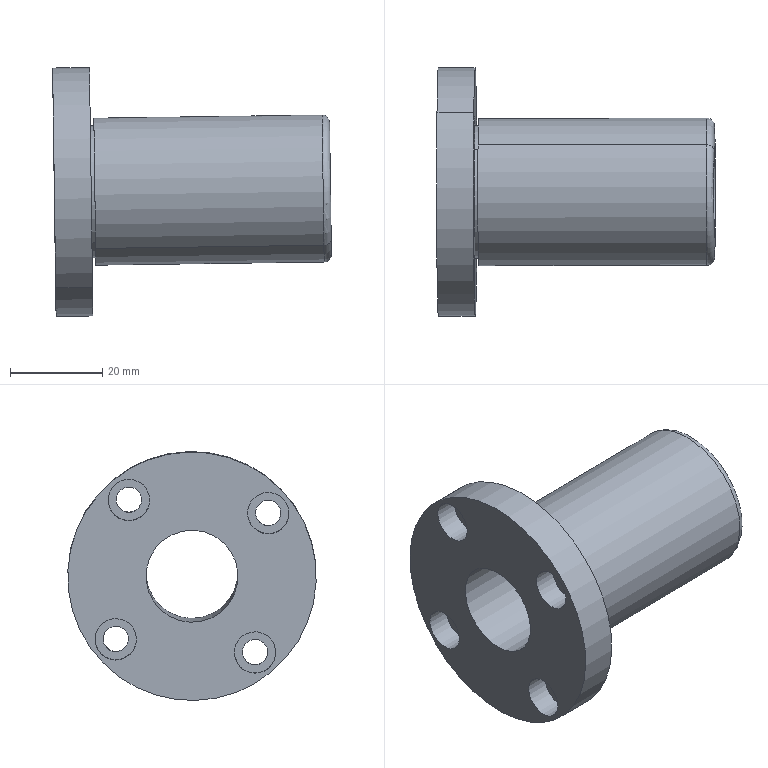Component | SolidWorks | DA-0220-LHFR20-1-15 | 1 solid | 34 faces | box 60.57 x 54 x 54.11 mm | volume 39543 mm3 | cylinder 24 | plane 8 | torus 2 | commonest cylinder face diameters 9 x8 5.5 x8 20 x2 28.8 x2 32 x2 54 x2
STEP:
#1=COLOUR_RGB('',0.7922,0.8196,0.9333);
#2=FILL_AREA_STYLE_COLOUR('',#1);
#3=FILL_AREA_STYLE('',(#2));
#4=SURFACE_STYLE_FILL_AREA(#3);
#5=SURFACE_SIDE_STYLE('',(#4));
#6=SURFACE_STYLE_USAGE(.BOTH.,#5);
#7=PRESENTATION_STYLE_ASSIGNMENT((#6));
#8=CARTESIAN_POINT('',(20.766,-3.293,-2.237));
#9=VERTEX_POINT('',#8);
#10=CARTESIAN_POINT('',(20.78,-4.096,-3.207));
#11=VERTEX_POINT('',#10);
#12=CARTESIAN_POINT('',(20.773,-3.694,-2.722));
#13=DIRECTION('',(-0.9999,-0.000404,-0.01395));
#14=DIRECTION('',(0.01101,-0.6374,-0.7704));
#15=AXIS2_PLACEMENT_3D('',#12,#13,#14);
#16=CIRCLE('',#15,0.6299);
#17=EDGE_CURVE('',#9,#11,#16,.T.);
#18=ORIENTED_EDGE('',*,*,#17,.F.);
#19=CARTESIAN_POINT('',(20.83,-3.333,-2.285));
#20=VERTEX_POINT('',#19);
#21=CARTESIAN_POINT('',(20.767,-3.333,-2.285));
#22=DIRECTION('',(0.008584,0.7705,-0.6374));
#23=DIRECTION('',(0.,0.6374,0.7705));
#24=AXIS2_PLACEMENT_3D('',#21,#22,#23);
#25=CIRCLE('',#24,0.06299);
#26=EDGE_CURVE('',#9,#20,#25,.T.);
#27=ORIENTED_EDGE('',*,*,#26,.T.);
#28=CARTESIAN_POINT('',(20.843,-4.056,-3.158));
#29=VERTEX_POINT('',#28);
#30=CARTESIAN_POINT('',(20.836,-3.694,-2.721));
#31=DIRECTION('',(0.9999,0.000404,0.01395));
#32=DIRECTION('',(0.01101,-0.6374,-0.7704));
#33=AXIS2_PLACEMENT_3D('',#30,#31,#32);
#34=CIRCLE('',#33,0.5669);
#35=EDGE_CURVE('',#29,#20,#34,.T.);
#36=ORIENTED_EDGE('',*,*,#35,.F.);
#37=CARTESIAN_POINT('',(20.78,-4.056,-3.159));
#38=DIRECTION('',(-0.008584,-0.7705,0.6374));
#39=DIRECTION('',(0.,-0.6374,-0.7705));
#40=AXIS2_PLACEMENT_3D('',#37,#38,#39);
#41=CIRCLE('',#40,0.06299);
#42=EDGE_CURVE('',#11,#29,#41,.T.);
#43=ORIENTED_EDGE('',*,*,#42,.F.);
#44=EDGE_LOOP('',(#18,#27,#36,#43));
#45=FACE_OUTER_BOUND('',#44,.T.);
#46=CARTESIAN_POINT('',(20.773,-3.694,-2.722));
#47=DIRECTION('',(0.9999,0.000404,0.01395));
#48=DIRECTION('',(0.01101,-0.6374,-0.7704));
#49=AXIS2_PLACEMENT_3D('',#46,#47,#48);
#50=TOROIDAL_SURFACE('',#49,0.5669,0.06299);
#51=ADVANCED_FACE('',(#45),#50,.T.);
#52=CARTESIAN_POINT('',(18.668,-3.269,-2.236));
#53=VERTEX_POINT('',#52);
#54=CARTESIAN_POINT('',(18.664,-3.043,-1.963));
#55=VERTEX_POINT('',#54);
#56=CARTESIAN_POINT('',(18.666,-3.156,-2.099));
#57=DIRECTION('',(-0.9999,-0.000404,-0.01395));
#58=DIRECTION('',(-0.01101,0.6374,0.7704));
#59=AXIS2_PLACEMENT_3D('',#56,#57,#58);
#60=CIRCLE('',#59,0.1772);
#61=EDGE_CURVE('',#53,#55,#60,.T.);
#62=ORIENTED_EDGE('',*,*,#61,.F.);
#63=CARTESIAN_POINT('',(18.467,-3.269,-2.239));
#64=VERTEX_POINT('',#63);
#65=CARTESIAN_POINT('',(18.467,-3.269,-2.239));
#66=DIRECTION('',(-0.9999,-0.000404,-0.01395));
#67=VECTOR('',#66,39.37);
#68=LINE('',#65,#67);
#69=EDGE_CURVE('',#53,#64,#68,.T.);
#70=ORIENTED_EDGE('',*,*,#69,.T.);
#71=CARTESIAN_POINT('',(18.463,-3.043,-1.966));
#72=VERTEX_POINT('',#71);
#73=CARTESIAN_POINT('',(18.465,-3.156,-2.102));
#74=DIRECTION('',(-0.9999,-0.000404,-0.01395));
#75=DIRECTION('',(-0.01101,0.6374,0.7704));
#76=AXIS2_PLACEMENT_3D('',#73,#74,#75);
#77=CIRCLE('',#76,0.1772);
#78=EDGE_CURVE('',#64,#72,#77,.T.);
#79=ORIENTED_EDGE('',*,*,#78,.T.);
#80=CARTESIAN_POINT('',(18.463,-3.043,-1.966));
#81=DIRECTION('',(-0.9999,-0.000404,-0.01395));
#82=VECTOR('',#81,39.37);
#83=LINE('',#80,#82);
#84=EDGE_CURVE('',#55,#72,#83,.T.);
#85=ORIENTED_EDGE('',*,*,#84,.F.);
#86=EDGE_LOOP('',(#62,#70,#79,#85));
#87=FACE_OUTER_BOUND('',#86,.T.);
#88=CARTESIAN_POINT('',(18.465,-3.156,-2.102));
#89=DIRECTION('',(-0.9999,-0.000404,-0.01395));
#90=DIRECTION('',(-0.01101,0.6374,0.7704));
#91=AXIS2_PLACEMENT_3D('',#88,#89,#90);
#92=CYLINDRICAL_SURFACE('',#91,0.1772);
#93=ADVANCED_FACE('',(#87),#92,.F.);
#94=CARTESIAN_POINT('',(18.779,-3.087,-2.014));
#95=VERTEX_POINT('',#94);
#96=CARTESIAN_POINT('',(18.781,-3.225,-2.181));
#97=VERTEX_POINT('',#96);
#98=CARTESIAN_POINT('',(18.78,-3.156,-2.098));
#99=DIRECTION('',(0.9999,0.000404,0.01395));
#100=DIRECTION('',(0.01101,-0.6374,-0.7704));
#101=AXIS2_PLACEMENT_3D('',#98,#99,#100);
#102=CIRCLE('',#101,0.1083);
#103=EDGE_CURVE('',#95,#97,#102,.T.);
#104=ORIENTED_EDGE('',*,*,#103,.T.);
#105=CARTESIAN_POINT('',(18.667,-3.225,-2.183));
#106=VERTEX_POINT('',#105);
#107=CARTESIAN_POINT('',(18.466,-3.225,-2.186));
#108=DIRECTION('',(-0.9999,-0.000404,-0.01395));
#109=VECTOR('',#108,39.37);
#110=LINE('',#107,#109);
#111=EDGE_CURVE('',#97,#106,#110,.T.);
#112=ORIENTED_EDGE('',*,*,#111,.T.);
#113=CARTESIAN_POINT('',(18.665,-3.087,-2.016));
#114=VERTEX_POINT('',#113);
#115=CARTESIAN_POINT('',(18.666,-3.156,-2.099));
#116=DIRECTION('',(-0.9999,-0.000404,-0.01395));
#117=DIRECTION('',(-0.01101,0.6374,0.7704));
#118=AXIS2_PLACEMENT_3D('',#115,#116,#117);
#119=CIRCLE('',#118,0.1083);
#120=EDGE_CURVE('',#106,#114,#119,.T.);
#121=ORIENTED_EDGE('',*,*,#120,.T.);
#122=CARTESIAN_POINT('',(18.464,-3.087,-2.019));
#123=DIRECTION('',(-0.9999,-0.000404,-0.01395));
#124=VECTOR('',#123,39.37);
#125=LINE('',#122,#124);
#126=EDGE_CURVE('',#95,#114,#125,.T.);
#127=ORIENTED_EDGE('',*,*,#126,.F.);
#128=EDGE_LOOP('',(#104,#112,#121,#127));
#129=FACE_OUTER_BOUND('',#128,.T.);
#130=CARTESIAN_POINT('',(18.465,-3.156,-2.102));
#131=DIRECTION('',(-0.9999,-0.000404,-0.01395));
#132=DIRECTION('',(-0.01101,0.6374,0.7704));
#133=AXIS2_PLACEMENT_3D('',#130,#131,#132);
#134=CYLINDRICAL_SURFACE('',#133,0.1083);
#135=ADVANCED_FACE('',(#129),#134,.F.);
#136=CARTESIAN_POINT('',(18.67,-4.46,-2.348));
#137=VERTEX_POINT('',#136);
#138=CARTESIAN_POINT('',(18.666,-4.235,-2.075));
#139=VERTEX_POINT('',#138);
#140=CARTESIAN_POINT('',(18.668,-4.348,-2.212));
#141=DIRECTION('',(-0.9999,-0.000404,-0.01395));
#142=DIRECTION('',(-0.01101,0.6374,0.7704));
#143=AXIS2_PLACEMENT_3D('',#140,#141,#142);
#144=CIRCLE('',#143,0.1772);
#145=EDGE_CURVE('',#137,#139,#144,.T.);
#146=ORIENTED_EDGE('',*,*,#145,.F.);
#147=CARTESIAN_POINT('',(18.469,-4.461,-2.351));
#148=VERTEX_POINT('',#147);
#149=CARTESIAN_POINT('',(18.469,-4.461,-2.351));
#150=DIRECTION('',(-0.9999,-0.000404,-0.01395));
#151=VECTOR('',#150,39.37);
#152=LINE('',#149,#151);
#153=EDGE_CURVE('',#137,#148,#152,.T.);
#154=ORIENTED_EDGE('',*,*,#153,.T.);
#155=CARTESIAN_POINT('',(18.465,-4.235,-2.078));
#156=VERTEX_POINT('',#155);
#157=CARTESIAN_POINT('',(18.467,-4.348,-2.215));
#158=DIRECTION('',(-0.9999,-0.000404,-0.01395));
#159=DIRECTION('',(-0.01101,0.6374,0.7704));
#160=AXIS2_PLACEMENT_3D('',#157,#158,#159);
#161=CIRCLE('',#160,0.1772);
#162=EDGE_CURVE('',#148,#156,#161,.T.);
#163=ORIENTED_EDGE('',*,*,#162,.T.);
#164=CARTESIAN_POINT('',(18.465,-4.235,-2.078));
#165=DIRECTION('',(-0.9999,-0.000404,-0.01395));
#166=VECTOR('',#165,39.37);
#167=LINE('',#164,#166);
#168=EDGE_CURVE('',#139,#156,#167,.T.);
#169=ORIENTED_EDGE('',*,*,#168,.F.);
#170=EDGE_LOOP('',(#146,#154,#163,#169));
#171=FACE_OUTER_BOUND('',#170,.T.);
#172=CARTESIAN_POINT('',(18.467,-4.348,-2.215));
#173=DIRECTION('',(-0.9999,-0.000404,-0.01395));
#174=DIRECTION('',(-0.01101,0.6374,0.7704));
#175=AXIS2_PLACEMENT_3D('',#172,#173,#174);
#176=CYLINDRICAL_SURFACE('',#175,0.1772);
#177=ADVANCED_FACE('',(#171),#176,.F.);
#178=CARTESIAN_POINT('',(18.781,-4.278,-2.127));
#179=VERTEX_POINT('',#178);
#180=CARTESIAN_POINT('',(18.783,-4.416,-2.294));
#181=VERTEX_POINT('',#180);
#182=CARTESIAN_POINT('',(18.782,-4.347,-2.21));
#183=DIRECTION('',(0.9999,0.000404,0.01395));
#184=DIRECTION('',(0.01101,-0.6374,-0.7704));
#185=AXIS2_PLACEMENT_3D('',#182,#183,#184);
#186=CIRCLE('',#185,0.1083);
#187=EDGE_CURVE('',#179,#181,#186,.T.);
#188=ORIENTED_EDGE('',*,*,#187,.T.);
#189=CARTESIAN_POINT('',(18.669,-4.417,-2.295));
#190=VERTEX_POINT('',#189);
#191=CARTESIAN_POINT('',(18.468,-4.417,-2.298));
#192=DIRECTION('',(-0.9999,-0.000404,-0.01395));
#193=VECTOR('',#192,39.37);
#194=LINE('',#191,#193);
#195=EDGE_CURVE('',#181,#190,#194,.T.);
#196=ORIENTED_EDGE('',*,*,#195,.T.);
#197=CARTESIAN_POINT('',(18.667,-4.278,-2.129));
#198=VERTEX_POINT('',#197);
#199=CARTESIAN_POINT('',(18.668,-4.348,-2.212));
#200=DIRECTION('',(-0.9999,-0.000404,-0.01395));
#201=DIRECTION('',(-0.01101,0.6374,0.7704));
#202=AXIS2_PLACEMENT_3D('',#199,#200,#201);
#203=CIRCLE('',#202,0.1083);
#204=EDGE_CURVE('',#190,#198,#203,.T.);
#205=ORIENTED_EDGE('',*,*,#204,.T.);
#206=CARTESIAN_POINT('',(18.466,-4.279,-2.131));
#207=DIRECTION('',(-0.9999,-0.000404,-0.01395));
#208=VECTOR('',#207,39.37);
#209=LINE('',#206,#208);
#210=EDGE_CURVE('',#179,#198,#209,.T.);
#211=ORIENTED_EDGE('',*,*,#210,.F.);
#212=EDGE_LOOP('',(#188,#196,#205,#211));
#213=FACE_OUTER_BOUND('',#212,.T.);
#214=CARTESIAN_POINT('',(18.467,-4.348,-2.215));
#215=DIRECTION('',(-0.9999,-0.000404,-0.01395));
#216=DIRECTION('',(-0.01101,0.6374,0.7704));
#217=AXIS2_PLACEMENT_3D('',#214,#215,#216);
#218=CYLINDRICAL_SURFACE('',#217,0.1083);
#219=ADVANCED_FACE('',(#213),#218,.F.);
#220=CARTESIAN_POINT('',(18.686,-4.348,-3.54));
#221=VERTEX_POINT('',#220);
#222=CARTESIAN_POINT('',(18.683,-4.122,-3.267));
#223=VERTEX_POINT('',#222);
#224=CARTESIAN_POINT('',(18.685,-4.235,-3.404));
#225=DIRECTION('',(-0.9999,-0.000404,-0.01395));
#226=DIRECTION('',(-0.01101,0.6374,0.7704));
#227=AXIS2_PLACEMENT_3D('',#224,#225,#226);
#228=CIRCLE('',#227,0.1772);
#229=EDGE_CURVE('',#221,#223,#228,.T.);
#230=ORIENTED_EDGE('',*,*,#229,.F.);
#231=CARTESIAN_POINT('',(18.486,-4.348,-3.543));
#232=VERTEX_POINT('',#231);
#233=CARTESIAN_POINT('',(18.486,-4.348,-3.543));
#234=DIRECTION('',(-0.9999,-0.000404,-0.01395));
#235=VECTOR('',#234,39.37);
#236=LINE('',#233,#235);
#237=EDGE_CURVE('',#221,#232,#236,.T.);
#238=ORIENTED_EDGE('',*,*,#237,.T.);
#239=CARTESIAN_POINT('',(18.482,-4.122,-3.27));
#240=VERTEX_POINT('',#239);
#241=CARTESIAN_POINT('',(18.484,-4.235,-3.406));
#242=DIRECTION('',(-0.9999,-0.000404,-0.01395));
#243=DIRECTION('',(-0.01101,0.6374,0.7704));
#244=AXIS2_PLACEMENT_3D('',#241,#242,#243);
#245=CIRCLE('',#244,0.1772);
#246=EDGE_CURVE('',#232,#240,#245,.T.);
#247=ORIENTED_EDGE('',*,*,#246,.T.);
#248=CARTESIAN_POINT('',(18.482,-4.122,-3.27));
#249=DIRECTION('',(-0.9999,-0.000404,-0.01395));
#250=VECTOR('',#249,39.37);
#251=LINE('',#248,#250);
#252=EDGE_CURVE('',#223,#240,#251,.T.);
#253=ORIENTED_EDGE('',*,*,#252,.F.);
#254=EDGE_LOOP('',(#230,#238,#247,#253));
#255=FACE_OUTER_BOUND('',#254,.T.);
#256=CARTESIAN_POINT('',(18.484,-4.235,-3.406));
#257=DIRECTION('',(-0.9999,-0.000404,-0.01395));
#258=DIRECTION('',(-0.01101,0.6374,0.7704));
#259=AXIS2_PLACEMENT_3D('',#256,#257,#258);
#260=CYLINDRICAL_SURFACE('',#259,0.1772);
#261=ADVANCED_FACE('',(#255),#260,.F.);
#262=CARTESIAN_POINT('',(18.797,-4.166,-3.319));
#263=VERTEX_POINT('',#262);
#264=CARTESIAN_POINT('',(18.8,-4.304,-3.485));
#265=VERTEX_POINT('',#264);
#266=CARTESIAN_POINT('',(18.799,-4.235,-3.402));
#267=DIRECTION('',(0.9999,0.000404,0.01395));
#268=DIRECTION('',(0.01101,-0.6374,-0.7704));
#269=AXIS2_PLACEMENT_3D('',#266,#267,#268);
#270=CIRCLE('',#269,0.1083);
#271=EDGE_CURVE('',#263,#265,#270,.T.);
#272=ORIENTED_EDGE('',*,*,#271,.T.);
#273=CARTESIAN_POINT('',(18.686,-4.304,-3.487));
#274=VERTEX_POINT('',#273);
#275=CARTESIAN_POINT('',(18.485,-4.304,-3.49));
#276=DIRECTION('',(-0.9999,-0.000404,-0.01395));
#277=VECTOR('',#276,39.37);
#278=LINE('',#275,#277);
#279=EDGE_CURVE('',#265,#274,#278,.T.);
#280=ORIENTED_EDGE('',*,*,#279,.T.);
#281=CARTESIAN_POINT('',(18.683,-4.166,-3.32));
#282=VERTEX_POINT('',#281);
#283=CARTESIAN_POINT('',(18.685,-4.235,-3.404));
#284=DIRECTION('',(-0.9999,-0.000404,-0.01395));
#285=DIRECTION('',(-0.01101,0.6374,0.7704));
#286=AXIS2_PLACEMENT_3D('',#283,#284,#285);
#287=CIRCLE('',#286,0.1083);
#288=EDGE_CURVE('',#274,#282,#287,.T.);
#289=ORIENTED_EDGE('',*,*,#288,.T.);
#290=CARTESIAN_POINT('',(18.483,-4.166,-3.323));
#291=DIRECTION('',(-0.9999,-0.000404,-0.01395));
#292=VECTOR('',#291,39.37);
#293=LINE('',#290,#292);
#294=EDGE_CURVE('',#263,#282,#293,.T.);
#295=ORIENTED_EDGE('',*,*,#294,.F.);
#296=EDGE_LOOP('',(#272,#280,#289,#295));
#297=FACE_OUTER_BOUND('',#296,.T.);
#298=CARTESIAN_POINT('',(18.484,-4.235,-3.406));
#299=DIRECTION('',(-0.9999,-0.000404,-0.01395));
#300=DIRECTION('',(-0.01101,0.6374,0.7704));
#301=AXIS2_PLACEMENT_3D('',#298,#299,#300);
#302=CYLINDRICAL_SURFACE('',#301,0.1083);
#303=ADVANCED_FACE('',(#297),#302,.F.);
#304=CARTESIAN_POINT('',(18.684,-3.156,-3.427));
#305=VERTEX_POINT('',#304);
#306=CARTESIAN_POINT('',(18.681,-2.93,-3.154));
#307=VERTEX_POINT('',#306);
#308=CARTESIAN_POINT('',(18.682,-3.043,-3.291));
#309=DIRECTION('',(-0.9999,-0.000404,-0.01395));
#310=DIRECTION('',(-0.01101,0.6374,0.7704));
#311=AXIS2_PLACEMENT_3D('',#308,#309,#310);
#312=CIRCLE('',#311,0.1772);
#313=EDGE_CURVE('',#305,#307,#312,.T.);
#314=ORIENTED_EDGE('',*,*,#313,.F.);
#315=CARTESIAN_POINT('',(18.484,-3.156,-3.43));
#316=VERTEX_POINT('',#315);
#317=CARTESIAN_POINT('',(18.484,-3.156,-3.43));
#318=DIRECTION('',(-0.9999,-0.000404,-0.01395));
#319=VECTOR('',#318,39.37);
#320=LINE('',#317,#319);
#321=EDGE_CURVE('',#305,#316,#320,.T.);
#322=ORIENTED_EDGE('',*,*,#321,.T.);
#323=CARTESIAN_POINT('',(18.48,-2.93,-3.157));
#324=VERTEX_POINT('',#323);
#325=CARTESIAN_POINT('',(18.482,-3.043,-3.294));
#326=DIRECTION('',(-0.9999,-0.000404,-0.01395));
#327=DIRECTION('',(-0.01101,0.6374,0.7704));
#328=AXIS2_PLACEMENT_3D('',#325,#326,#327);
#329=CIRCLE('',#328,0.1772);
#330=EDGE_CURVE('',#316,#324,#329,.T.);
#331=ORIENTED_EDGE('',*,*,#330,.T.);
#332=CARTESIAN_POINT('',(18.48,-2.93,-3.157));
#333=DIRECTION('',(-0.9999,-0.000404,-0.01395));
#334=VECTOR('',#333,39.37);
#335=LINE('',#332,#334);
#336=EDGE_CURVE('',#307,#324,#335,.T.);
#337=ORIENTED_EDGE('',*,*,#336,.F.);
#338=EDGE_LOOP('',(#314,#322,#331,#337));
#339=FACE_OUTER_BOUND('',#338,.T.);
#340=CARTESIAN_POINT('',(18.482,-3.043,-3.294));
#341=DIRECTION('',(-0.9999,-0.000404,-0.01395));
#342=DIRECTION('',(-0.01101,0.6374,0.7704));
#343=AXIS2_PLACEMENT_3D('',#340,#341,#342);
#344=CYLINDRICAL_SURFACE('',#343,0.1772);
#345=ADVANCED_FACE('',(#339),#344,.F.);
#346=CARTESIAN_POINT('',(18.795,-2.974,-3.206));
#347=VERTEX_POINT('',#346);
#348=CARTESIAN_POINT('',(18.798,-3.112,-3.373));
#349=VERTEX_POINT('',#348);
#350=CARTESIAN_POINT('',(18.797,-3.043,-3.289));
#351=DIRECTION('',(0.9999,0.000404,0.01395));
#352=DIRECTION('',(0.01101,-0.6374,-0.7704));
#353=AXIS2_PLACEMENT_3D('',#350,#351,#352);
#354=CIRCLE('',#353,0.1083);
#355=EDGE_CURVE('',#347,#349,#354,.T.);
#356=ORIENTED_EDGE('',*,*,#355,.T.);
#357=CARTESIAN_POINT('',(18.684,-3.112,-3.374));
#358=VERTEX_POINT('',#357);
#359=CARTESIAN_POINT('',(18.483,-3.112,-3.377));
#360=DIRECTION('',(-0.9999,-0.000404,-0.01395));
#361=VECTOR('',#360,39.37);
#362=LINE('',#359,#361);
#363=EDGE_CURVE('',#349,#358,#362,.T.);
#364=ORIENTED_EDGE('',*,*,#363,.T.);
#365=CARTESIAN_POINT('',(18.681,-2.974,-3.208));
#366=VERTEX_POINT('',#365);
#367=CARTESIAN_POINT('',(18.682,-3.043,-3.291));
#368=DIRECTION('',(-0.9999,-0.000404,-0.01395));
#369=DIRECTION('',(-0.01101,0.6374,0.7704));
#370=AXIS2_PLACEMENT_3D('',#367,#368,#369);
#371=CIRCLE('',#370,0.1083);
#372=EDGE_CURVE('',#358,#366,#371,.T.);
#373=ORIENTED_EDGE('',*,*,#372,.T.);
#374=CARTESIAN_POINT('',(18.481,-2.974,-3.21));
#375=DIRECTION('',(-0.9999,-0.000404,-0.01395));
#376=VECTOR('',#375,39.37);
#377=LINE('',#374,#376);
#378=EDGE_CURVE('',#347,#366,#377,.T.);
#379=ORIENTED_EDGE('',*,*,#378,.F.);
#380=EDGE_LOOP('',(#356,#364,#373,#379));
#381=FACE_OUTER_BOUND('',#380,.T.);
#382=CARTESIAN_POINT('',(18.482,-3.043,-3.294));
#383=DIRECTION('',(-0.9999,-0.000404,-0.01395));
#384=DIRECTION('',(-0.01101,0.6374,0.7704));
#385=AXIS2_PLACEMENT_3D('',#382,#383,#384);
#386=CYLINDRICAL_SURFACE('',#385,0.1083);
#387=ADVANCED_FACE('',(#381),#386,.F.);
#388=CARTESIAN_POINT('',(20.841,-3.945,-3.025));
#389=VERTEX_POINT('',#388);
#390=CARTESIAN_POINT('',(20.832,-3.443,-2.418));
#391=VERTEX_POINT('',#390);
#392=CARTESIAN_POINT('',(20.836,-3.694,-2.721));
#393=DIRECTION('',(-0.9999,-0.000404,-0.01395));
#394=DIRECTION('',(-0.01101,0.6374,0.7704));
#395=AXIS2_PLACEMENT_3D('',#392,#393,#394);
#396=CIRCLE('',#395,0.3937);
#397=EDGE_CURVE('',#389,#391,#396,.T.);
#398=ORIENTED_EDGE('',*,*,#397,.F.);
#399=CARTESIAN_POINT('',(18.479,-3.946,-3.058));
#400=VERTEX_POINT('',#399);
#401=CARTESIAN_POINT('',(18.479,-3.946,-3.058));
#402=DIRECTION('',(-0.9999,-0.000404,-0.01395));
#403=VECTOR('',#402,39.37);
#404=LINE('',#401,#403);
#405=EDGE_CURVE('',#389,#400,#404,.T.);
#406=ORIENTED_EDGE('',*,*,#405,.T.);
#407=CARTESIAN_POINT('',(18.47,-3.444,-2.451));
#408=VERTEX_POINT('',#407);
#409=CARTESIAN_POINT('',(18.474,-3.695,-2.754));
#410=DIRECTION('',(-0.9999,-0.000404,-0.01395));
#411=DIRECTION('',(-0.01101,0.6374,0.7704));
#412=AXIS2_PLACEMENT_3D('',#409,#410,#411);
#413=CIRCLE('',#412,0.3937);
#414=EDGE_CURVE('',#400,#408,#413,.T.);
#415=ORIENTED_EDGE('',*,*,#414,.T.);
#416=CARTESIAN_POINT('',(18.47,-3.444,-2.451));
#417=DIRECTION('',(-0.9999,-0.000404,-0.01395));
#418=VECTOR('',#417,39.37);
#419=LINE('',#416,#418);
#420=EDGE_CURVE('',#391,#408,#419,.T.);
#421=ORIENTED_EDGE('',*,*,#420,.F.);
#422=EDGE_LOOP('',(#398,#406,#415,#421));
#423=FACE_OUTER_BOUND('',#422,.T.);
#424=CARTESIAN_POINT('',(18.474,-3.695,-2.754));
#425=DIRECTION('',(-0.9999,-0.000404,-0.01395));
#426=DIRECTION('',(-0.01101,0.6374,0.7704));
#427=AXIS2_PLACEMENT_3D('',#424,#425,#426);
#428=CYLINDRICAL_SURFACE('',#427,0.3937);
#429=ADVANCED_FACE('',(#423),#428,.F.);
#430=CARTESIAN_POINT('',(18.796,-4.057,-3.187));
#431=VERTEX_POINT('',#430);
#432=CARTESIAN_POINT('',(18.783,-3.334,-2.313));
#433=VERTEX_POINT('',#432);
#434=CARTESIAN_POINT('',(18.789,-3.695,-2.75));
#435=DIRECTION('',(0.9999,0.000404,0.01395));
#436=DIRECTION('',(0.01101,-0.6374,-0.7704));
#437=AXIS2_PLACEMENT_3D('',#434,#435,#436);
#438=CIRCLE('',#437,0.5669);
#439=EDGE_CURVE('',#431,#433,#438,.T.);
#440=ORIENTED_EDGE('',*,*,#439,.T.);
#441=CARTESIAN_POINT('',(18.815,-3.334,-2.313));
#442=VERTEX_POINT('',#441);
#443=CARTESIAN_POINT('',(18.468,-3.334,-2.317));
#444=DIRECTION('',(0.9999,0.000404,0.01395));
#445=VECTOR('',#444,39.37);
#446=LINE('',#443,#445);
#447=EDGE_CURVE('',#433,#442,#446,.T.);
#448=ORIENTED_EDGE('',*,*,#447,.T.);
#449=CARTESIAN_POINT('',(18.827,-4.057,-3.186));
#450=VERTEX_POINT('',#449);
#451=CARTESIAN_POINT('',(18.821,-3.695,-2.749));
#452=DIRECTION('',(0.9999,0.000404,0.01395));
#453=DIRECTION('',(0.01101,-0.6374,-0.7704));
#454=AXIS2_PLACEMENT_3D('',#451,#452,#453);
#455=CIRCLE('',#454,0.5669);
#456=EDGE_CURVE('',#450,#442,#455,.T.);
#457=ORIENTED_EDGE('',*,*,#456,.F.);
#458=CARTESIAN_POINT('',(18.481,-4.057,-3.191));
#459=DIRECTION('',(0.9999,0.000404,0.01395));
#460=VECTOR('',#459,39.37);
#461=LINE('',#458,#460);
#462=EDGE_CURVE('',#431,#450,#461,.T.);
#463=ORIENTED_EDGE('',*,*,#462,.F.);
#464=EDGE_LOOP('',(#440,#448,#457,#463));
#465=FACE_OUTER_BOUND('',#464,.T.);
#466=CARTESIAN_POINT('',(18.474,-3.695,-2.754));
#467=DIRECTION('',(0.9999,0.000404,0.01395));
#468=DIRECTION('',(0.01101,-0.6374,-0.7704));
#469=AXIS2_PLACEMENT_3D('',#466,#467,#468);
#470=CYLINDRICAL_SURFACE('',#469,0.5669);
#471=ADVANCED_FACE('',(#465),#470,.T.);
#472=CARTESIAN_POINT('',(18.828,-4.097,-3.235));
#473=VERTEX_POINT('',#472);
#474=CARTESIAN_POINT('',(18.814,-3.294,-2.264));
#475=VERTEX_POINT('',#474);
#476=CARTESIAN_POINT('',(18.821,-3.695,-2.749));
#477=DIRECTION('',(0.9999,0.000404,0.01395));
#478=DIRECTION('',(0.01101,-0.6374,-0.7704));
#479=AXIS2_PLACEMENT_3D('',#476,#477,#478);
#480=CIRCLE('',#479,0.6299);
#481=EDGE_CURVE('',#473,#475,#480,.T.);
#482=ORIENTED_EDGE('',*,*,#481,.T.);
#483=CARTESIAN_POINT('',(18.468,-3.294,-2.269));
#484=DIRECTION('',(0.9999,0.000404,0.01395));
#485=VECTOR('',#484,39.37);
#486=LINE('',#483,#485);
#487=EDGE_CURVE('',#475,#9,#486,.T.);
#488=ORIENTED_EDGE('',*,*,#487,.T.);
#489=ORIENTED_EDGE('',*,*,#17,.T.);
#490=CARTESIAN_POINT('',(18.481,-4.097,-3.24));
#491=DIRECTION('',(0.9999,0.000404,0.01395));
#492=VECTOR('',#491,39.37);
#493=LINE('',#490,#492);
#494=EDGE_CURVE('',#473,#11,#493,.T.);
#495=ORIENTED_EDGE('',*,*,#494,.F.);
#496=EDGE_LOOP('',(#482,#488,#489,#495));
#497=FACE_OUTER_BOUND('',#496,.T.);
#498=CARTESIAN_POINT('',(18.474,-3.695,-2.754));
#499=DIRECTION('',(0.9999,0.000404,0.01395));
#500=DIRECTION('',(0.01101,-0.6374,-0.7704));
#501=AXIS2_PLACEMENT_3D('',#498,#499,#500);
#502=CYLINDRICAL_SURFACE('',#501,0.6299);
#503=ADVANCED_FACE('',(#497),#502,.T.);
#504=CARTESIAN_POINT('',(18.486,-4.373,-3.573));
#505=VERTEX_POINT('',#504);
#506=CARTESIAN_POINT('',(18.463,-3.018,-1.935));
#507=VERTEX_POINT('',#506);
#508=CARTESIAN_POINT('',(18.474,-3.695,-2.754));
#509=DIRECTION('',(0.9999,0.000404,0.01395));
#510=DIRECTION('',(0.01101,-0.6374,-0.7704));
#511=AXIS2_PLACEMENT_3D('',#508,#509,#510);
#512=CIRCLE('',#511,1.063);
#513=EDGE_CURVE('',#505,#507,#512,.T.);
#514=ORIENTED_EDGE('',*,*,#513,.T.);
#515=CARTESIAN_POINT('',(18.778,-3.018,-1.931));
#516=VERTEX_POINT('',#515);
#517=CARTESIAN_POINT('',(18.463,-3.018,-1.935));
#518=DIRECTION('',(0.9999,0.000404,0.01395));
#519=VECTOR('',#518,39.37);
#520=LINE('',#517,#519);
#521=EDGE_CURVE('',#507,#516,#520,.T.);
#522=ORIENTED_EDGE('',*,*,#521,.T.);
#523=CARTESIAN_POINT('',(18.801,-4.373,-3.569));
#524=VERTEX_POINT('',#523);
#525=CARTESIAN_POINT('',(18.789,-3.695,-2.75));
#526=DIRECTION('',(0.9999,0.000404,0.01395));
#527=DIRECTION('',(0.01101,-0.6374,-0.7704));
#528=AXIS2_PLACEMENT_3D('',#525,#526,#527);
#529=CIRCLE('',#528,1.063);
#530=EDGE_CURVE('',#524,#516,#529,.T.);
#531=ORIENTED_EDGE('',*,*,#530,.F.);
#532=CARTESIAN_POINT('',(18.486,-4.373,-3.573));
#533=DIRECTION('',(0.9999,0.000404,0.01395));
#534=VECTOR('',#533,39.37);
#535=LINE('',#532,#534);
#536=EDGE_CURVE('',#505,#524,#535,.T.);
#537=ORIENTED_EDGE('',*,*,#536,.F.);
#538=EDGE_LOOP('',(#514,#522,#531,#537));
#539=FACE_OUTER_BOUND('',#538,.T.);
#540=CARTESIAN_POINT('',(18.474,-3.695,-2.754));
#541=DIRECTION('',(0.9999,0.000404,0.01395));
#542=DIRECTION('',(0.01101,-0.6374,-0.7704));
#543=AXIS2_PLACEMENT_3D('',#540,#541,#542);
#544=CYLINDRICAL_SURFACE('',#543,1.063);
#545=ADVANCED_FACE('',(#539),#544,.T.);
#546=ORIENTED_EDGE('',*,*,#521,.F.);
#547=CARTESIAN_POINT('',(18.474,-3.695,-2.754));
#548=DIRECTION('',(0.9999,0.000404,0.01395));
#549=DIRECTION('',(0.01101,-0.6374,-0.7704));
#550=AXIS2_PLACEMENT_3D('',#547,#548,#549);
#551=CIRCLE('',#550,1.063);
#552=EDGE_CURVE('',#507,#505,#551,.T.);
#553=ORIENTED_EDGE('',*,*,#552,.T.);
#554=ORIENTED_EDGE('',*,*,#536,.T.);
#555=CARTESIAN_POINT('',(18.789,-3.695,-2.75));
#556=DIRECTION('',(0.9999,0.000404,0.01395));
#557=DIRECTION('',(0.01101,-0.6374,-0.7704));
#558=AXIS2_PLACEMENT_3D('',#555,#556,#557);
#559=CIRCLE('',#558,1.063);
#560=EDGE_CURVE('',#516,#524,#559,.T.);
#561=ORIENTED_EDGE('',*,*,#560,.F.);
#562=EDGE_LOOP('',(#546,#553,#554,#561));
#563=FACE_OUTER_BOUND('',#562,.T.);
#564=CARTESIAN_POINT('',(18.474,-3.695,-2.754));
#565=DIRECTION('',(0.9999,0.000404,0.01395));
#566=DIRECTION('',(0.01101,-0.6374,-0.7704));
#567=AXIS2_PLACEMENT_3D('',#564,#565,#566);
#568=CYLINDRICAL_SURFACE('',#567,1.063);
#569=ADVANCED_FACE('',(#563),#568,.T.);
#570=CARTESIAN_POINT('',(18.465,-3.156,-2.102));
#571=DIRECTION('',(-0.9999,-0.000404,-0.01395));
#572=DIRECTION('',(-0.01101,0.6374,0.7704));
#573=AXIS2_PLACEMENT_3D('',#570,#571,#572);
#574=CIRCLE('',#573,0.1772);
#575=EDGE_CURVE('',#72,#64,#574,.T.);
#576=ORIENTED_EDGE('',*,*,#575,.F.);
#577=ORIENTED_EDGE('',*,*,#78,.F.);
#578=EDGE_LOOP('',(#576,#577));
#579=FACE_BOUND('',#578,.T.);
#580=CARTESIAN_POINT('',(18.467,-4.348,-2.215));
#581=DIRECTION('',(-0.9999,-0.000404,-0.01395));
#582=DIRECTION('',(-0.01101,0.6374,0.7704));
#583=AXIS2_PLACEMENT_3D('',#580,#581,#582);
#584=CIRCLE('',#583,0.1772);
#585=EDGE_CURVE('',#156,#148,#584,.T.);
#586=ORIENTED_EDGE('',*,*,#585,.F.);
#587=ORIENTED_EDGE('',*,*,#162,.F.);
#588=EDGE_LOOP('',(#586,#587));
#589=FACE_BOUND('',#588,.T.);
#590=CARTESIAN_POINT('',(18.484,-4.235,-3.406));
#591=DIRECTION('',(-0.9999,-0.000404,-0.01395));
#592=DIRECTION('',(-0.01101,0.6374,0.7704));
#593=AXIS2_PLACEMENT_3D('',#590,#591,#592);
#594=CIRCLE('',#593,0.1772);
#595=EDGE_CURVE('',#240,#232,#594,.T.);
#596=ORIENTED_EDGE('',*,*,#595,.F.);
#597=ORIENTED_EDGE('',*,*,#246,.F.);
#598=EDGE_LOOP('',(#596,#597));
#599=FACE_BOUND('',#598,.T.);
#600=CARTESIAN_POINT('',(18.482,-3.043,-3.294));
#601=DIRECTION('',(-0.9999,-0.000404,-0.01395));
#602=DIRECTION('',(-0.01101,0.6374,0.7704));
#603=AXIS2_PLACEMENT_3D('',#600,#601,#602);
#604=CIRCLE('',#603,0.1772);
#605=EDGE_CURVE('',#324,#316,#604,.T.);
#606=ORIENTED_EDGE('',*,*,#605,.F.);
#607=ORIENTED_EDGE('',*,*,#330,.F.);
#608=EDGE_LOOP('',(#606,#607));
#609=FACE_BOUND('',#608,.T.);
#610=CARTESIAN_POINT('',(18.474,-3.695,-2.754));
#611=DIRECTION('',(-0.9999,-0.000404,-0.01395));
#612=DIRECTION('',(-0.01101,0.6374,0.7704));
#613=AXIS2_PLACEMENT_3D('',#610,#611,#612);
#614=CIRCLE('',#613,0.3937);
#615=EDGE_CURVE('',#408,#400,#614,.T.);
#616=ORIENTED_EDGE('',*,*,#615,.F.);
#617=ORIENTED_EDGE('',*,*,#414,.F.);
#618=EDGE_LOOP('',(#616,#617));
#619=FACE_BOUND('',#618,.T.);
#620=ORIENTED_EDGE('',*,*,#513,.F.);
#621=ORIENTED_EDGE('',*,*,#552,.F.);
#622=EDGE_LOOP('',(#620,#621));
#623=FACE_OUTER_BOUND('',#622,.T.);
#624=CARTESIAN_POINT('',(18.484,-2.876,-3.432));
#625=DIRECTION('',(-0.9999,-0.000404,-0.01395));
#626=DIRECTION('',(-0.01101,0.6374,0.7704));
#627=AXIS2_PLACEMENT_3D('',#624,#625,#626);
#628=PLANE('',#627);
#629=ADVANCED_FACE('',(#579,#589,#599,#609,#619,#623),#628,.T.);
#630=ORIENTED_EDGE('',*,*,#35,.T.);
#631=CARTESIAN_POINT('',(20.836,-3.694,-2.721));
#632=DIRECTION('',(0.9999,0.000404,0.01395));
#633=DIRECTION('',(0.01101,-0.6374,-0.7704));
#634=AXIS2_PLACEMENT_3D('',#631,#632,#633);
#635=CIRCLE('',#634,0.5669);
#636=EDGE_CURVE('',#20,#29,#635,.T.);
#637=ORIENTED_EDGE('',*,*,#636,.T.);
#638=EDGE_LOOP('',(#630,#637));
#639=FACE_OUTER_BOUND('',#638,.T.);
#640=CARTESIAN_POINT('',(20.836,-3.694,-2.721));
#641=DIRECTION('',(-0.9999,-0.000404,-0.01395));
#642=DIRECTION('',(-0.01101,0.6374,0.7704));
#643=AXIS2_PLACEMENT_3D('',#640,#641,#642);
#644=CIRCLE('',#643,0.3937);
#645=EDGE_CURVE('',#391,#389,#644,.T.);
#646=ORIENTED_EDGE('',*,*,#645,.T.);
#647=ORIENTED_EDGE('',*,*,#397,.T.);
#648=EDGE_LOOP('',(#646,#647));
#649=FACE_BOUND('',#648,.T.);
#650=CARTESIAN_POINT('',(20.836,-3.694,-2.721));
#651=DIRECTION('',(0.9999,0.000404,0.01395));
#652=DIRECTION('',(0.01101,-0.6374,-0.7704));
#653=AXIS2_PLACEMENT_3D('',#650,#651,#652);
#654=PLANE('',#653);
#655=ADVANCED_FACE('',(#639,#649),#654,.T.);
#656=ORIENTED_EDGE('',*,*,#487,.F.);
#657=CARTESIAN_POINT('',(18.821,-3.695,-2.749));
#658=DIRECTION('',(0.9999,0.000404,0.01395));
#659=DIRECTION('',(0.01101,-0.6374,-0.7704));
#660=AXIS2_PLACEMENT_3D('',#657,#658,#659);
#661=CIRCLE('',#660,0.6299);
#662=EDGE_CURVE('',#475,#473,#661,.T.);
#663=ORIENTED_EDGE('',*,*,#662,.T.);
#664=ORIENTED_EDGE('',*,*,#494,.T.);
#665=CARTESIAN_POINT('',(20.773,-3.694,-2.722));
#666=DIRECTION('',(-0.9999,-0.000404,-0.01395));
#667=DIRECTION('',(0.01101,-0.6374,-0.7704));
#668=AXIS2_PLACEMENT_3D('',#665,#666,#667);
#669=CIRCLE('',#668,0.6299);
#670=EDGE_CURVE('',#11,#9,#669,.T.);
#671=ORIENTED_EDGE('',*,*,#670,.T.);
#672=EDGE_LOOP('',(#656,#663,#664,#671));
#673=FACE_OUTER_BOUND('',#672,.T.);
#674=CARTESIAN_POINT('',(18.474,-3.695,-2.754));
#675=DIRECTION('',(0.9999,0.000404,0.01395));
#676=DIRECTION('',(0.01101,-0.6374,-0.7704));
#677=AXIS2_PLACEMENT_3D('',#674,#675,#676);
#678=CYLINDRICAL_SURFACE('',#677,0.6299);
#679=ADVANCED_FACE('',(#673),#678,.T.);
#680=ORIENTED_EDGE('',*,*,#456,.T.);
#681=CARTESIAN_POINT('',(18.821,-3.695,-2.749));
#682=DIRECTION('',(0.9999,0.000404,0.01395));
#683=DIRECTION('',(0.01101,-0.6374,-0.7704));
#684=AXIS2_PLACEMENT_3D('',#681,#682,#683);
#685=CIRCLE('',#684,0.5669);
#686=EDGE_CURVE('',#442,#450,#685,.T.);
#687=ORIENTED_EDGE('',*,*,#686,.T.);
#688=EDGE_LOOP('',(#680,#687));
#689=FACE_BOUND('',#688,.T.);
#690=ORIENTED_EDGE('',*,*,#481,.F.);
#691=ORIENTED_EDGE('',*,*,#662,.F.);
#692=EDGE_LOOP('',(#690,#691));
#693=FACE_OUTER_BOUND('',#692,.T.);
#694=CARTESIAN_POINT('',(18.826,-3.21,-3.151));
#695=DIRECTION('',(-0.9999,-0.000404,-0.01395));
#696=DIRECTION('',(-0.01101,0.6374,0.7704));
#697=AXIS2_PLACEMENT_3D('',#694,#695,#696);
#698=PLANE('',#697);
#699=ADVANCED_FACE('',(#689,#693),#698,.T.);
#700=ORIENTED_EDGE('',*,*,#447,.F.);
#701=CARTESIAN_POINT('',(18.789,-3.695,-2.75));
#702=DIRECTION('',(0.9999,0.000404,0.01395));
#703=DIRECTION('',(0.01101,-0.6374,-0.7704));
#704=AXIS2_PLACEMENT_3D('',#701,#702,#703);
#705=CIRCLE('',#704,0.5669);
#706=EDGE_CURVE('',#433,#431,#705,.T.);
#707=ORIENTED_EDGE('',*,*,#706,.T.);
#708=ORIENTED_EDGE('',*,*,#462,.T.);
#709=ORIENTED_EDGE('',*,*,#686,.F.);
#710=EDGE_LOOP('',(#700,#707,#708,#709));
#711=FACE_OUTER_BOUND('',#710,.T.);
#712=CARTESIAN_POINT('',(18.474,-3.695,-2.754));
#713=DIRECTION('',(0.9999,0.000404,0.01395));
#714=DIRECTION('',(0.01101,-0.6374,-0.7704));
#715=AXIS2_PLACEMENT_3D('',#712,#713,#714);
#716=CYLINDRICAL_SURFACE('',#715,0.5669);
#717=ADVANCED_FACE('',(#711),#716,.T.);
#718=ORIENTED_EDGE('',*,*,#103,.F.);
#719=CARTESIAN_POINT('',(18.78,-3.156,-2.098));
#720=DIRECTION('',(0.9999,0.000404,0.01395));
#721=DIRECTION('',(0.01101,-0.6374,-0.7704));
#722=AXIS2_PLACEMENT_3D('',#719,#720,#721);
#723=CIRCLE('',#722,0.1083);
#724=EDGE_CURVE('',#97,#95,#723,.T.);
#725=ORIENTED_EDGE('',*,*,#724,.F.);
#726=EDGE_LOOP('',(#718,#725));
#727=FACE_BOUND('',#726,.T.);
#728=ORIENTED_EDGE('',*,*,#187,.F.);
#729=CARTESIAN_POINT('',(18.782,-4.347,-2.21));
#730=DIRECTION('',(0.9999,0.000404,0.01395));
#731=DIRECTION('',(0.01101,-0.6374,-0.7704));
#732=AXIS2_PLACEMENT_3D('',#729,#730,#731);
#733=CIRCLE('',#732,0.1083);
#734=EDGE_CURVE('',#181,#179,#733,.T.);
#735=ORIENTED_EDGE('',*,*,#734,.F.);
#736=EDGE_LOOP('',(#728,#735));
#737=FACE_BOUND('',#736,.T.);
#738=ORIENTED_EDGE('',*,*,#271,.F.);
#739=CARTESIAN_POINT('',(18.799,-4.235,-3.402));
#740=DIRECTION('',(0.9999,0.000404,0.01395));
#741=DIRECTION('',(0.01101,-0.6374,-0.7704));
#742=AXIS2_PLACEMENT_3D('',#739,#740,#741);
#743=CIRCLE('',#742,0.1083);
#744=EDGE_CURVE('',#265,#263,#743,.T.);
#745=ORIENTED_EDGE('',*,*,#744,.F.);
#746=EDGE_LOOP('',(#738,#745));
#747=FACE_BOUND('',#746,.T.);
#748=ORIENTED_EDGE('',*,*,#355,.F.);
#749=CARTESIAN_POINT('',(18.797,-3.043,-3.289));
#750=DIRECTION('',(0.9999,0.000404,0.01395));
#751=DIRECTION('',(0.01101,-0.6374,-0.7704));
#752=AXIS2_PLACEMENT_3D('',#749,#750,#751);
#753=CIRCLE('',#752,0.1083);
#754=EDGE_CURVE('',#349,#347,#753,.T.);
#755=ORIENTED_EDGE('',*,*,#754,.F.);
#756=EDGE_LOOP('',(#748,#755));
#757=FACE_BOUND('',#756,.T.);
#758=ORIENTED_EDGE('',*,*,#530,.T.);
#759=ORIENTED_EDGE('',*,*,#560,.T.);
#760=EDGE_LOOP('',(#758,#759));
#761=FACE_OUTER_BOUND('',#760,.T.);
#762=ORIENTED_EDGE('',*,*,#439,.F.);
#763=ORIENTED_EDGE('',*,*,#706,.F.);
#764=EDGE_LOOP('',(#762,#763));
#765=FACE_BOUND('',#764,.T.);
#766=CARTESIAN_POINT('',(18.794,-3.258,-3.111));
#767=DIRECTION('',(0.9999,0.000404,0.01395));
#768=DIRECTION('',(0.01101,-0.6374,-0.7704));
#769=AXIS2_PLACEMENT_3D('',#766,#767,#768);
#770=PLANE('',#769);
#771=ADVANCED_FACE('',(#727,#737,#747,#757,#761,#765),#770,.T.);
#772=ORIENTED_EDGE('',*,*,#405,.F.);
#773=ORIENTED_EDGE('',*,*,#645,.F.);
#774=ORIENTED_EDGE('',*,*,#420,.T.);
#775=ORIENTED_EDGE('',*,*,#615,.T.);
#776=EDGE_LOOP('',(#772,#773,#774,#775));
#777=FACE_OUTER_BOUND('',#776,.T.);
#778=CARTESIAN_POINT('',(18.474,-3.695,-2.754));
#779=DIRECTION('',(-0.9999,-0.000404,-0.01395));
#780=DIRECTION('',(-0.01101,0.6374,0.7704));
#781=AXIS2_PLACEMENT_3D('',#778,#779,#780);
#782=CYLINDRICAL_SURFACE('',#781,0.3937);
#783=ADVANCED_FACE('',(#777),#782,.F.);
#784=ORIENTED_EDGE('',*,*,#363,.F.);
#785=ORIENTED_EDGE('',*,*,#754,.T.);
#786=ORIENTED_EDGE('',*,*,#378,.T.);
#787=CARTESIAN_POINT('',(18.682,-3.043,-3.291));
#788=DIRECTION('',(-0.9999,-0.000404,-0.01395));
#789=DIRECTION('',(-0.01101,0.6374,0.7704));
#790=AXIS2_PLACEMENT_3D('',#787,#788,#789);
#791=CIRCLE('',#790,0.1083);
#792=EDGE_CURVE('',#366,#358,#791,.T.);
#793=ORIENTED_EDGE('',*,*,#792,.T.);
#794=EDGE_LOOP('',(#784,#785,#786,#793));
#795=FACE_OUTER_BOUND('',#794,.T.);
#796=CARTESIAN_POINT('',(18.482,-3.043,-3.294));
#797=DIRECTION('',(-0.9999,-0.000404,-0.01395));
#798=DIRECTION('',(-0.01101,0.6374,0.7704));
#799=AXIS2_PLACEMENT_3D('',#796,#797,#798);
#800=CYLINDRICAL_SURFACE('',#799,0.1083);
#801=ADVANCED_FACE('',(#795),#800,.F.);
#802=ORIENTED_EDGE('',*,*,#792,.F.);
#803=ORIENTED_EDGE('',*,*,#372,.F.);
#804=EDGE_LOOP('',(#802,#803));
#805=FACE_BOUND('',#804,.T.);
#806=CARTESIAN_POINT('',(18.682,-3.043,-3.291));
#807=DIRECTION('',(-0.9999,-0.000404,-0.01395));
#808=DIRECTION('',(-0.01101,0.6374,0.7704));
#809=AXIS2_PLACEMENT_3D('',#806,#807,#808);
#810=CIRCLE('',#809,0.1772);
#811=EDGE_CURVE('',#307,#305,#810,.T.);
#812=ORIENTED_EDGE('',*,*,#811,.T.);
#813=ORIENTED_EDGE('',*,*,#313,.T.);
#814=EDGE_LOOP('',(#812,#813));
#815=FACE_OUTER_BOUND('',#814,.T.);
#816=CARTESIAN_POINT('',(18.683,-2.96,-3.36));
#817=DIRECTION('',(0.9999,0.000404,0.01395));
#818=DIRECTION('',(0.01101,-0.6374,-0.7704));
#819=AXIS2_PLACEMENT_3D('',#816,#817,#818);
#820=PLANE('',#819);
#821=ADVANCED_FACE('',(#805,#815),#820,.F.);
#822=ORIENTED_EDGE('',*,*,#321,.F.);
#823=ORIENTED_EDGE('',*,*,#811,.F.);
#824=ORIENTED_EDGE('',*,*,#336,.T.);
#825=ORIENTED_EDGE('',*,*,#605,.T.);
#826=EDGE_LOOP('',(#822,#823,#824,#825));
#827=FACE_OUTER_BOUND('',#826,.T.);
#828=CARTESIAN_POINT('',(18.482,-3.043,-3.294));
#829=DIRECTION('',(-0.9999,-0.000404,-0.01395));
#830=DIRECTION('',(-0.01101,0.6374,0.7704));
#831=AXIS2_PLACEMENT_3D('',#828,#829,#830);
#832=CYLINDRICAL_SURFACE('',#831,0.1772);
#833=ADVANCED_FACE('',(#827),#832,.F.);
#834=ORIENTED_EDGE('',*,*,#279,.F.);
#835=ORIENTED_EDGE('',*,*,#744,.T.);
#836=ORIENTED_EDGE('',*,*,#294,.T.);
#837=CARTESIAN_POINT('',(18.685,-4.235,-3.404));
#838=DIRECTION('',(-0.9999,-0.000404,-0.01395));
#839=DIRECTION('',(-0.01101,0.6374,0.7704));
#840=AXIS2_PLACEMENT_3D('',#837,#838,#839);
#841=CIRCLE('',#840,0.1083);
#842=EDGE_CURVE('',#282,#274,#841,.T.);
#843=ORIENTED_EDGE('',*,*,#842,.T.);
#844=EDGE_LOOP('',(#834,#835,#836,#843));
#845=FACE_OUTER_BOUND('',#844,.T.);
#846=CARTESIAN_POINT('',(18.484,-4.235,-3.406));
#847=DIRECTION('',(-0.9999,-0.000404,-0.01395));
#848=DIRECTION('',(-0.01101,0.6374,0.7704));
#849=AXIS2_PLACEMENT_3D('',#846,#847,#848);
#850=CYLINDRICAL_SURFACE('',#849,0.1083);
#851=ADVANCED_FACE('',(#845),#850,.F.);
#852=ORIENTED_EDGE('',*,*,#842,.F.);
#853=ORIENTED_EDGE('',*,*,#288,.F.);
#854=EDGE_LOOP('',(#852,#853));
#855=FACE_BOUND('',#854,.T.);
#856=CARTESIAN_POINT('',(18.685,-4.235,-3.404));
#857=DIRECTION('',(-0.9999,-0.000404,-0.01395));
#858=DIRECTION('',(-0.01101,0.6374,0.7704));
#859=AXIS2_PLACEMENT_3D('',#856,#857,#858);
#860=CIRCLE('',#859,0.1772);
#861=EDGE_CURVE('',#223,#221,#860,.T.);
#862=ORIENTED_EDGE('',*,*,#861,.T.);
#863=ORIENTED_EDGE('',*,*,#229,.T.);
#864=EDGE_LOOP('',(#862,#863));
#865=FACE_OUTER_BOUND('',#864,.T.);
#866=CARTESIAN_POINT('',(18.685,-4.151,-3.473));
#867=DIRECTION('',(0.9999,0.000404,0.01395));
#868=DIRECTION('',(0.01101,-0.6374,-0.7704));
#869=AXIS2_PLACEMENT_3D('',#866,#867,#868);
#870=PLANE('',#869);
#871=ADVANCED_FACE('',(#855,#865),#870,.F.);
#872=ORIENTED_EDGE('',*,*,#237,.F.);
#873=ORIENTED_EDGE('',*,*,#861,.F.);
#874=ORIENTED_EDGE('',*,*,#252,.T.);
#875=ORIENTED_EDGE('',*,*,#595,.T.);
#876=EDGE_LOOP('',(#872,#873,#874,#875));
#877=FACE_OUTER_BOUND('',#876,.T.);
#878=CARTESIAN_POINT('',(18.484,-4.235,-3.406));
#879=DIRECTION('',(-0.9999,-0.000404,-0.01395));
#880=DIRECTION('',(-0.01101,0.6374,0.7704));
#881=AXIS2_PLACEMENT_3D('',#878,#879,#880);
#882=CYLINDRICAL_SURFACE('',#881,0.1772);
#883=ADVANCED_FACE('',(#877),#882,.F.);
#884=ORIENTED_EDGE('',*,*,#195,.F.);
#885=ORIENTED_EDGE('',*,*,#734,.T.);
#886=ORIENTED_EDGE('',*,*,#210,.T.);
#887=CARTESIAN_POINT('',(18.668,-4.348,-2.212));
#888=DIRECTION('',(-0.9999,-0.000404,-0.01395));
#889=DIRECTION('',(-0.01101,0.6374,0.7704));
#890=AXIS2_PLACEMENT_3D('',#887,#888,#889);
#891=CIRCLE('',#890,0.1083);
#892=EDGE_CURVE('',#198,#190,#891,.T.);
#893=ORIENTED_EDGE('',*,*,#892,.T.);
#894=EDGE_LOOP('',(#884,#885,#886,#893));
#895=FACE_OUTER_BOUND('',#894,.T.);
#896=CARTESIAN_POINT('',(18.467,-4.348,-2.215));
#897=DIRECTION('',(-0.9999,-0.000404,-0.01395));
#898=DIRECTION('',(-0.01101,0.6374,0.7704));
#899=AXIS2_PLACEMENT_3D('',#896,#897,#898);
#900=CYLINDRICAL_SURFACE('',#899,0.1083);
#901=ADVANCED_FACE('',(#895),#900,.F.);
#902=ORIENTED_EDGE('',*,*,#892,.F.);
#903=ORIENTED_EDGE('',*,*,#204,.F.);
#904=EDGE_LOOP('',(#902,#903));
#905=FACE_BOUND('',#904,.T.);
#906=CARTESIAN_POINT('',(18.668,-4.348,-2.212));
#907=DIRECTION('',(-0.9999,-0.000404,-0.01395));
#908=DIRECTION('',(-0.01101,0.6374,0.7704));
#909=AXIS2_PLACEMENT_3D('',#906,#907,#908);
#910=CIRCLE('',#909,0.1772);
#911=EDGE_CURVE('',#139,#137,#910,.T.);
#912=ORIENTED_EDGE('',*,*,#911,.T.);
#913=ORIENTED_EDGE('',*,*,#145,.T.);
#914=EDGE_LOOP('',(#912,#913));
#915=FACE_OUTER_BOUND('',#914,.T.);
#916=CARTESIAN_POINT('',(18.669,-4.264,-2.281));
#917=DIRECTION('',(0.9999,0.000404,0.01395));
#918=DIRECTION('',(0.01101,-0.6374,-0.7704));
#919=AXIS2_PLACEMENT_3D('',#916,#917,#918);
#920=PLANE('',#919);
#921=ADVANCED_FACE('',(#905,#915),#920,.F.);
#922=ORIENTED_EDGE('',*,*,#153,.F.);
#923=ORIENTED_EDGE('',*,*,#911,.F.);
#924=ORIENTED_EDGE('',*,*,#168,.T.);
#925=ORIENTED_EDGE('',*,*,#585,.T.);
#926=EDGE_LOOP('',(#922,#923,#924,#925));
#927=FACE_OUTER_BOUND('',#926,.T.);
#928=CARTESIAN_POINT('',(18.467,-4.348,-2.215));
#929=DIRECTION('',(-0.9999,-0.000404,-0.01395));
#930=DIRECTION('',(-0.01101,0.6374,0.7704));
#931=AXIS2_PLACEMENT_3D('',#928,#929,#930);
#932=CYLINDRICAL_SURFACE('',#931,0.1772);
#933=ADVANCED_FACE('',(#927),#932,.F.);
#934=ORIENTED_EDGE('',*,*,#111,.F.);
#935=ORIENTED_EDGE('',*,*,#724,.T.);
#936=ORIENTED_EDGE('',*,*,#126,.T.);
#937=CARTESIAN_POINT('',(18.666,-3.156,-2.099));
#938=DIRECTION('',(-0.9999,-0.000404,-0.01395));
#939=DIRECTION('',(-0.01101,0.6374,0.7704));
#940=AXIS2_PLACEMENT_3D('',#937,#938,#939);
#941=CIRCLE('',#940,0.1083);
#942=EDGE_CURVE('',#114,#106,#941,.T.);
#943=ORIENTED_EDGE('',*,*,#942,.T.);
#944=EDGE_LOOP('',(#934,#935,#936,#943));
#945=FACE_OUTER_BOUND('',#944,.T.);
#946=CARTESIAN_POINT('',(18.465,-3.156,-2.102));
#947=DIRECTION('',(-0.9999,-0.000404,-0.01395));
#948=DIRECTION('',(-0.01101,0.6374,0.7704));
#949=AXIS2_PLACEMENT_3D('',#946,#947,#948);
#950=CYLINDRICAL_SURFACE('',#949,0.1083);
#951=ADVANCED_FACE('',(#945),#950,.F.);
#952=ORIENTED_EDGE('',*,*,#942,.F.);
#953=ORIENTED_EDGE('',*,*,#120,.F.);
#954=EDGE_LOOP('',(#952,#953));
#955=FACE_BOUND('',#954,.T.);
#956=CARTESIAN_POINT('',(18.666,-3.156,-2.099));
#957=DIRECTION('',(-0.9999,-0.000404,-0.01395));
#958=DIRECTION('',(-0.01101,0.6374,0.7704));
#959=AXIS2_PLACEMENT_3D('',#956,#957,#958);
#960=CIRCLE('',#959,0.1772);
#961=EDGE_CURVE('',#55,#53,#960,.T.);
#962=ORIENTED_EDGE('',*,*,#961,.T.);
#963=ORIENTED_EDGE('',*,*,#61,.T.);
#964=EDGE_LOOP('',(#962,#963));
#965=FACE_OUTER_BOUND('',#964,.T.);
#966=CARTESIAN_POINT('',(18.667,-3.072,-2.168));
#967=DIRECTION('',(0.9999,0.000404,0.01395));
#968=DIRECTION('',(0.01101,-0.6374,-0.7704));
#969=AXIS2_PLACEMENT_3D('',#966,#967,#968);
#970=PLANE('',#969);
#971=ADVANCED_FACE('',(#955,#965),#970,.F.);
#972=ORIENTED_EDGE('',*,*,#69,.F.);
#973=ORIENTED_EDGE('',*,*,#961,.F.);
#974=ORIENTED_EDGE('',*,*,#84,.T.);
#975=ORIENTED_EDGE('',*,*,#575,.T.);
#976=EDGE_LOOP('',(#972,#973,#974,#975));
#977=FACE_OUTER_BOUND('',#976,.T.);
#978=CARTESIAN_POINT('',(18.465,-3.156,-2.102));
#979=DIRECTION('',(-0.9999,-0.000404,-0.01395));
#980=DIRECTION('',(-0.01101,0.6374,0.7704));
#981=AXIS2_PLACEMENT_3D('',#978,#979,#980);
#982=CYLINDRICAL_SURFACE('',#981,0.1772);
#983=ADVANCED_FACE('',(#977),#982,.F.);
#984=ORIENTED_EDGE('',*,*,#26,.F.);
#985=ORIENTED_EDGE('',*,*,#670,.F.);
#986=ORIENTED_EDGE('',*,*,#42,.T.);
#987=ORIENTED_EDGE('',*,*,#636,.F.);
#988=EDGE_LOOP('',(#984,#985,#986,#987));
#989=FACE_OUTER_BOUND('',#988,.T.);
#990=CARTESIAN_POINT('',(20.773,-3.694,-2.722));
#991=DIRECTION('',(0.9999,0.000404,0.01395));
#992=DIRECTION('',(0.01101,-0.6374,-0.7704));
#993=AXIS2_PLACEMENT_3D('',#990,#991,#992);
#994=TOROIDAL_SURFACE('',#993,0.5669,0.06299);
#995=ADVANCED_FACE('',(#989),#994,.T.);
#996=CLOSED_SHELL('',(#51,#93,#135,#177,#219,#261,#303,#345,#387,#429,#471,#503,#545,#569,#629,#655,#679,#699,#717,#771,#783,#801,#821,#833,#851,#871,#883,#901,#921,#933,#951,#971,#983,#995));
#997=MANIFOLD_SOLID_BREP('',#996);
#998=STYLED_ITEM('',(#7),#997);
#999=PRESENTATION_LAYER_ASSIGNMENT('','',(#998));
#1000=(LENGTH_UNIT()NAMED_UNIT(*)SI_UNIT($,.METRE.));
#1001=LENGTH_MEASURE_WITH_UNIT(LENGTH_MEASURE(0.0254),#1000);
#1002=DIMENSIONAL_EXPONENTS(1.,0.,0.,0.,0.,0.,0.);
#1003=(CONVERSION_BASED_UNIT('',#1001)LENGTH_UNIT()NAMED_UNIT(#1002));
#1004=UNCERTAINTY_MEASURE_WITH_UNIT(LENGTH_MEASURE(0.00001),#1003,'','');
#1005=(NAMED_UNIT(*)PLANE_ANGLE_UNIT()SI_UNIT($,.RADIAN.));
#1006=(NAMED_UNIT(*)SI_UNIT($,.STERADIAN.)SOLID_ANGLE_UNIT());
#1007=(GEOMETRIC_REPRESENTATION_CONTEXT(3)GLOBAL_UNCERTAINTY_ASSIGNED_CONTEXT((#1004))GLOBAL_UNIT_ASSIGNED_CONTEXT((#1003,#1005,#1006))REPRESENTATION_CONTEXT('',''));
#1008=MECHANICAL_DESIGN_GEOMETRIC_PRESENTATION_REPRESENTATION('',(#998),#1007);
#1009=CARTESIAN_POINT('',(0.,0.,0.));
#1010=DIRECTION('',(0.,0.,1.));
#1011=DIRECTION('',(1.,0.,0.));
#1012=AXIS2_PLACEMENT_3D('',#1009,#1010,#1011);
#1013=(LENGTH_UNIT()NAMED_UNIT(*)SI_UNIT($,.METRE.));
#1014=LENGTH_MEASURE_WITH_UNIT(LENGTH_MEASURE(0.0254),#1013);
#1015=DIMENSIONAL_EXPONENTS(1.,0.,0.,0.,0.,0.,0.);
#1016=(CONVERSION_BASED_UNIT('',#1014)LENGTH_UNIT()NAMED_UNIT(#1015));
#1017=UNCERTAINTY_MEASURE_WITH_UNIT(LENGTH_MEASURE(0.00001),#1016,'','');
#1018=(NAMED_UNIT(*)PLANE_ANGLE_UNIT()SI_UNIT($,.RADIAN.));
#1019=(NAMED_UNIT(*)SI_UNIT($,.STERADIAN.)SOLID_ANGLE_UNIT());
#1020=(GEOMETRIC_REPRESENTATION_CONTEXT(3)GLOBAL_UNCERTAINTY_ASSIGNED_CONTEXT((#1017))GLOBAL_UNIT_ASSIGNED_CONTEXT((#1016,#1018,#1019))REPRESENTATION_CONTEXT('',''));
#1021=ADVANCED_BREP_SHAPE_REPRESENTATION('',(#997,#1012),#1020);